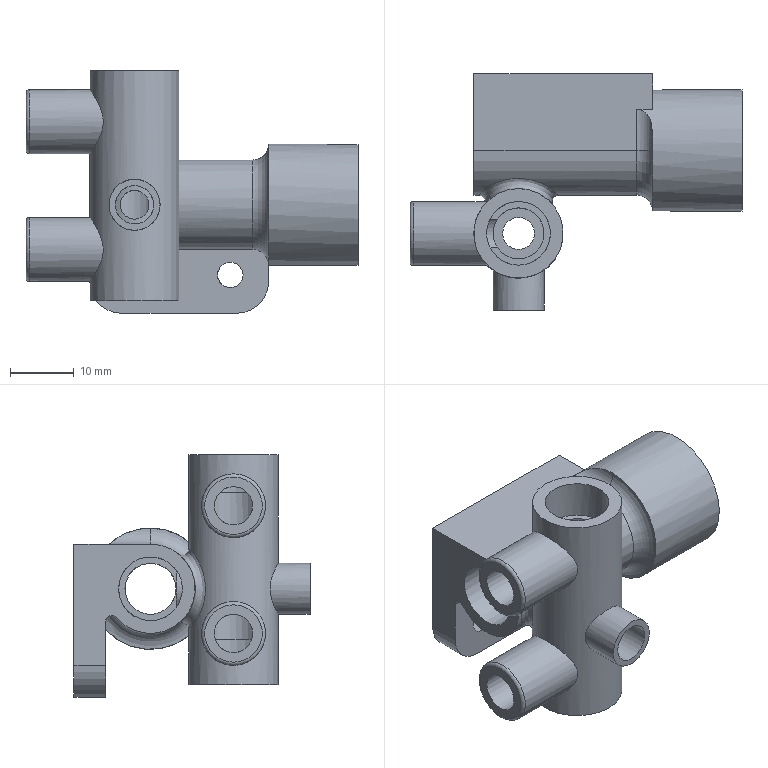Component | NX | OUTER_CASING_TUBE | 1 solid | 49 faces | volume 13021 mm3 | cylinder 26 | plane 19 | torus 3 | spline 1 | commonest cylinder face diameters 10 x7 8 x5 14 x4 6 x3 5 x2 4 x2 1.861 x1 19 x1